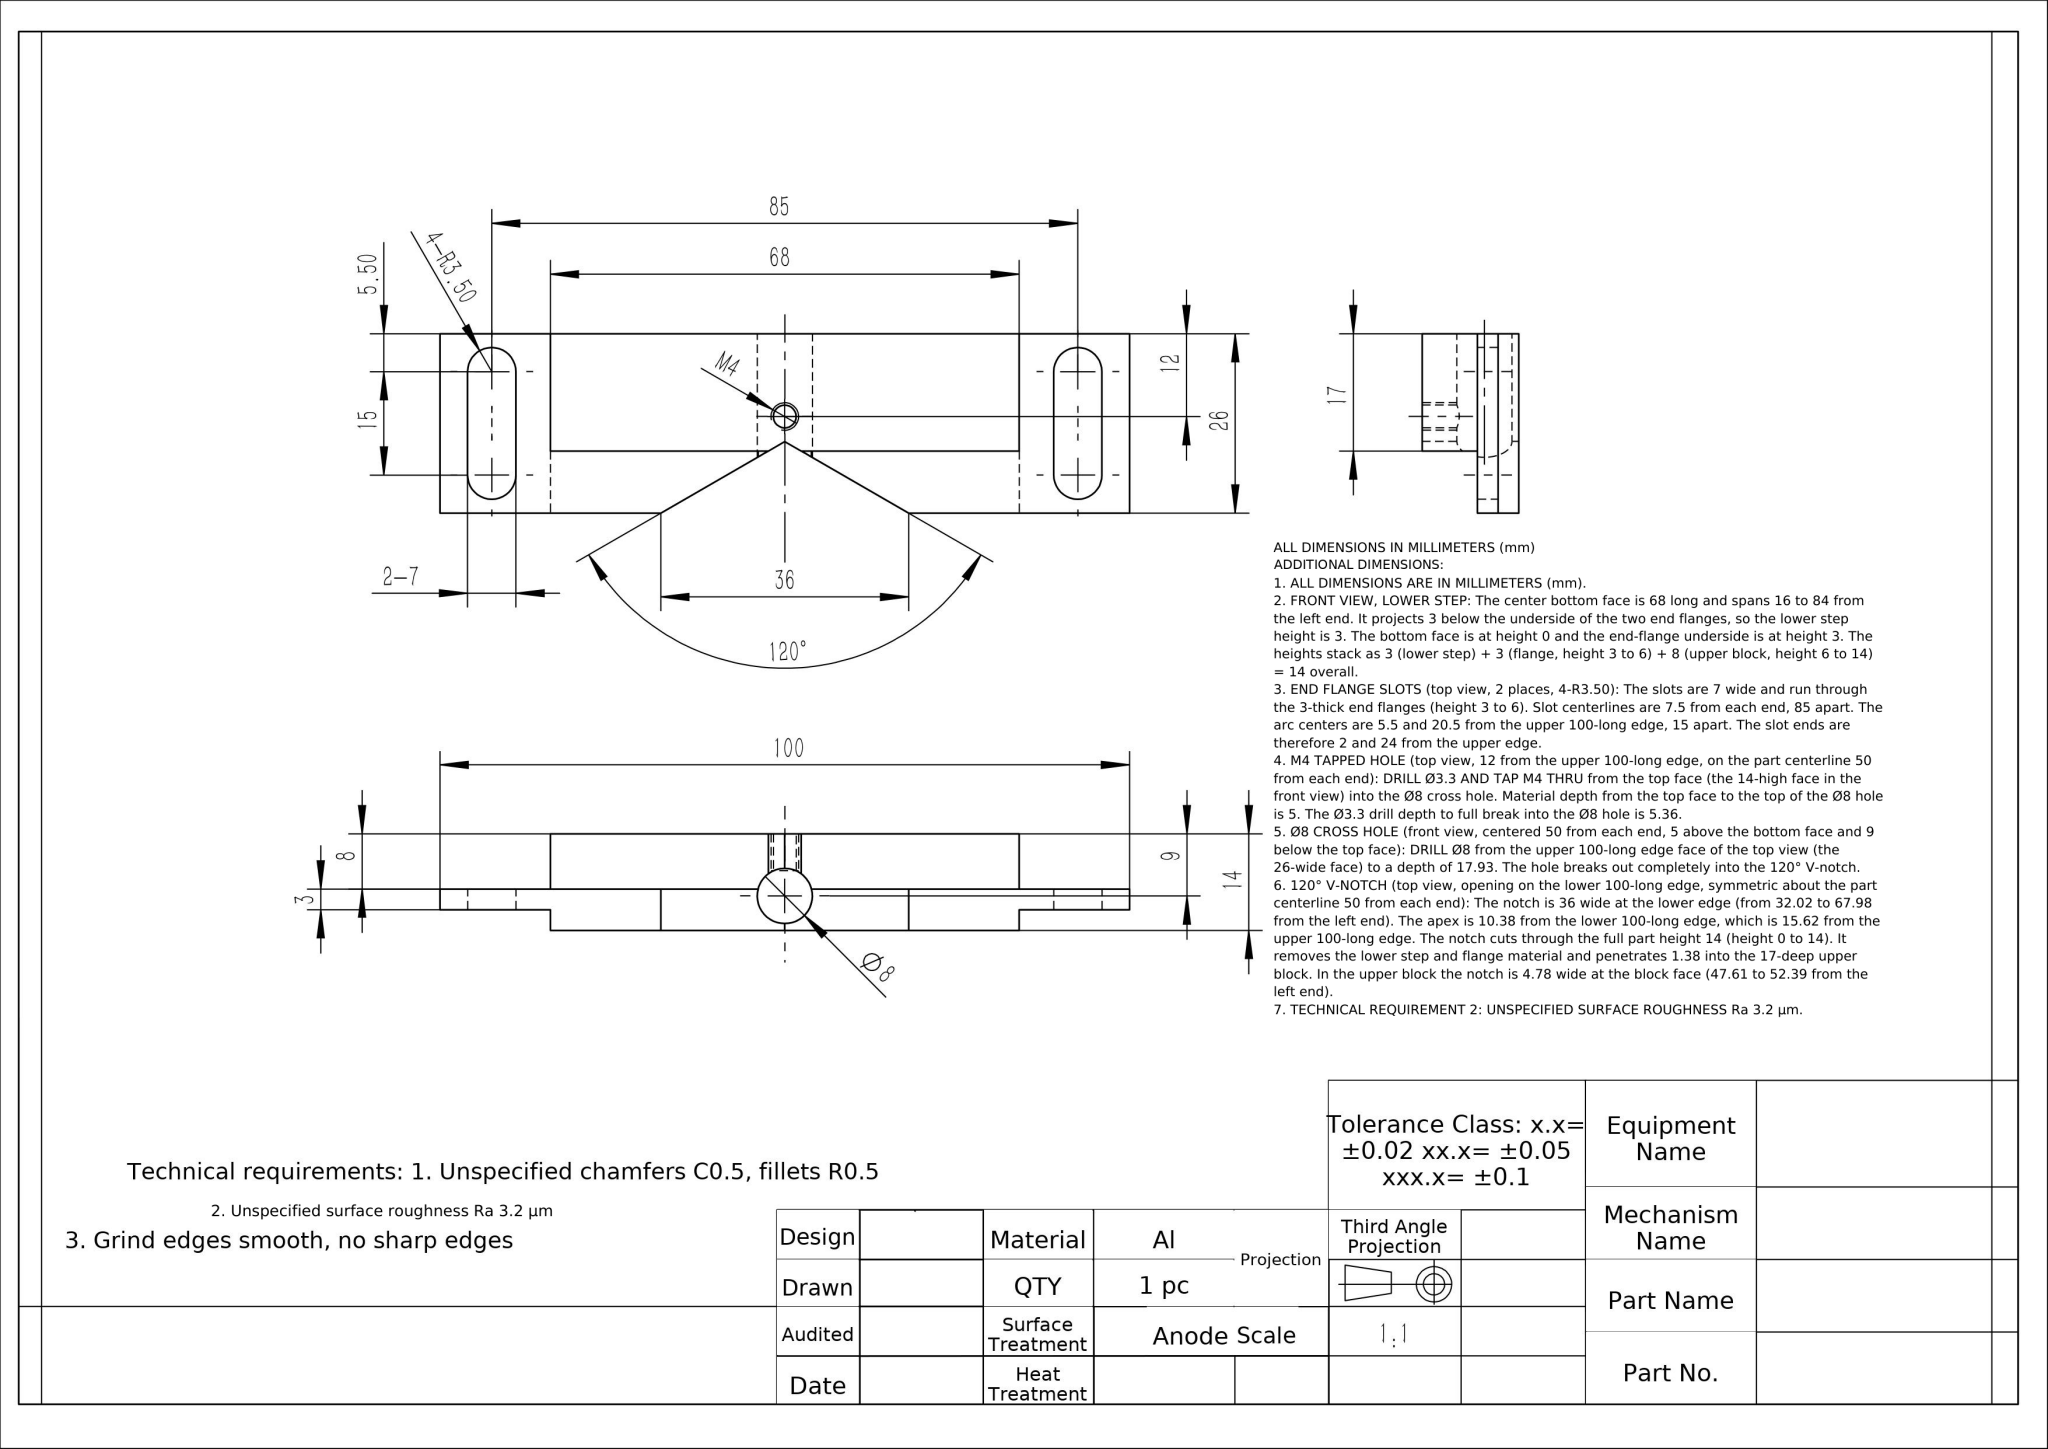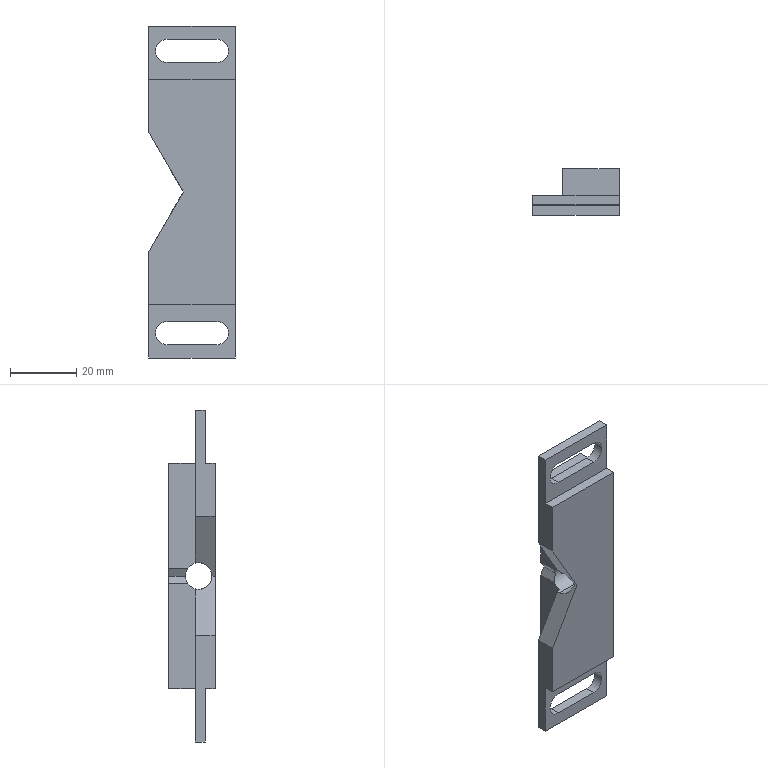Part | NX | mm | Dual-Slot Latch Mounting Block | 1 solid | 33 faces | box 26 x 14 x 100 mm | volume 19469 mm3 | plane 25 | cylinder 8 | commonest cylinder face diameters 7 x4 3.3 x2 8 x2